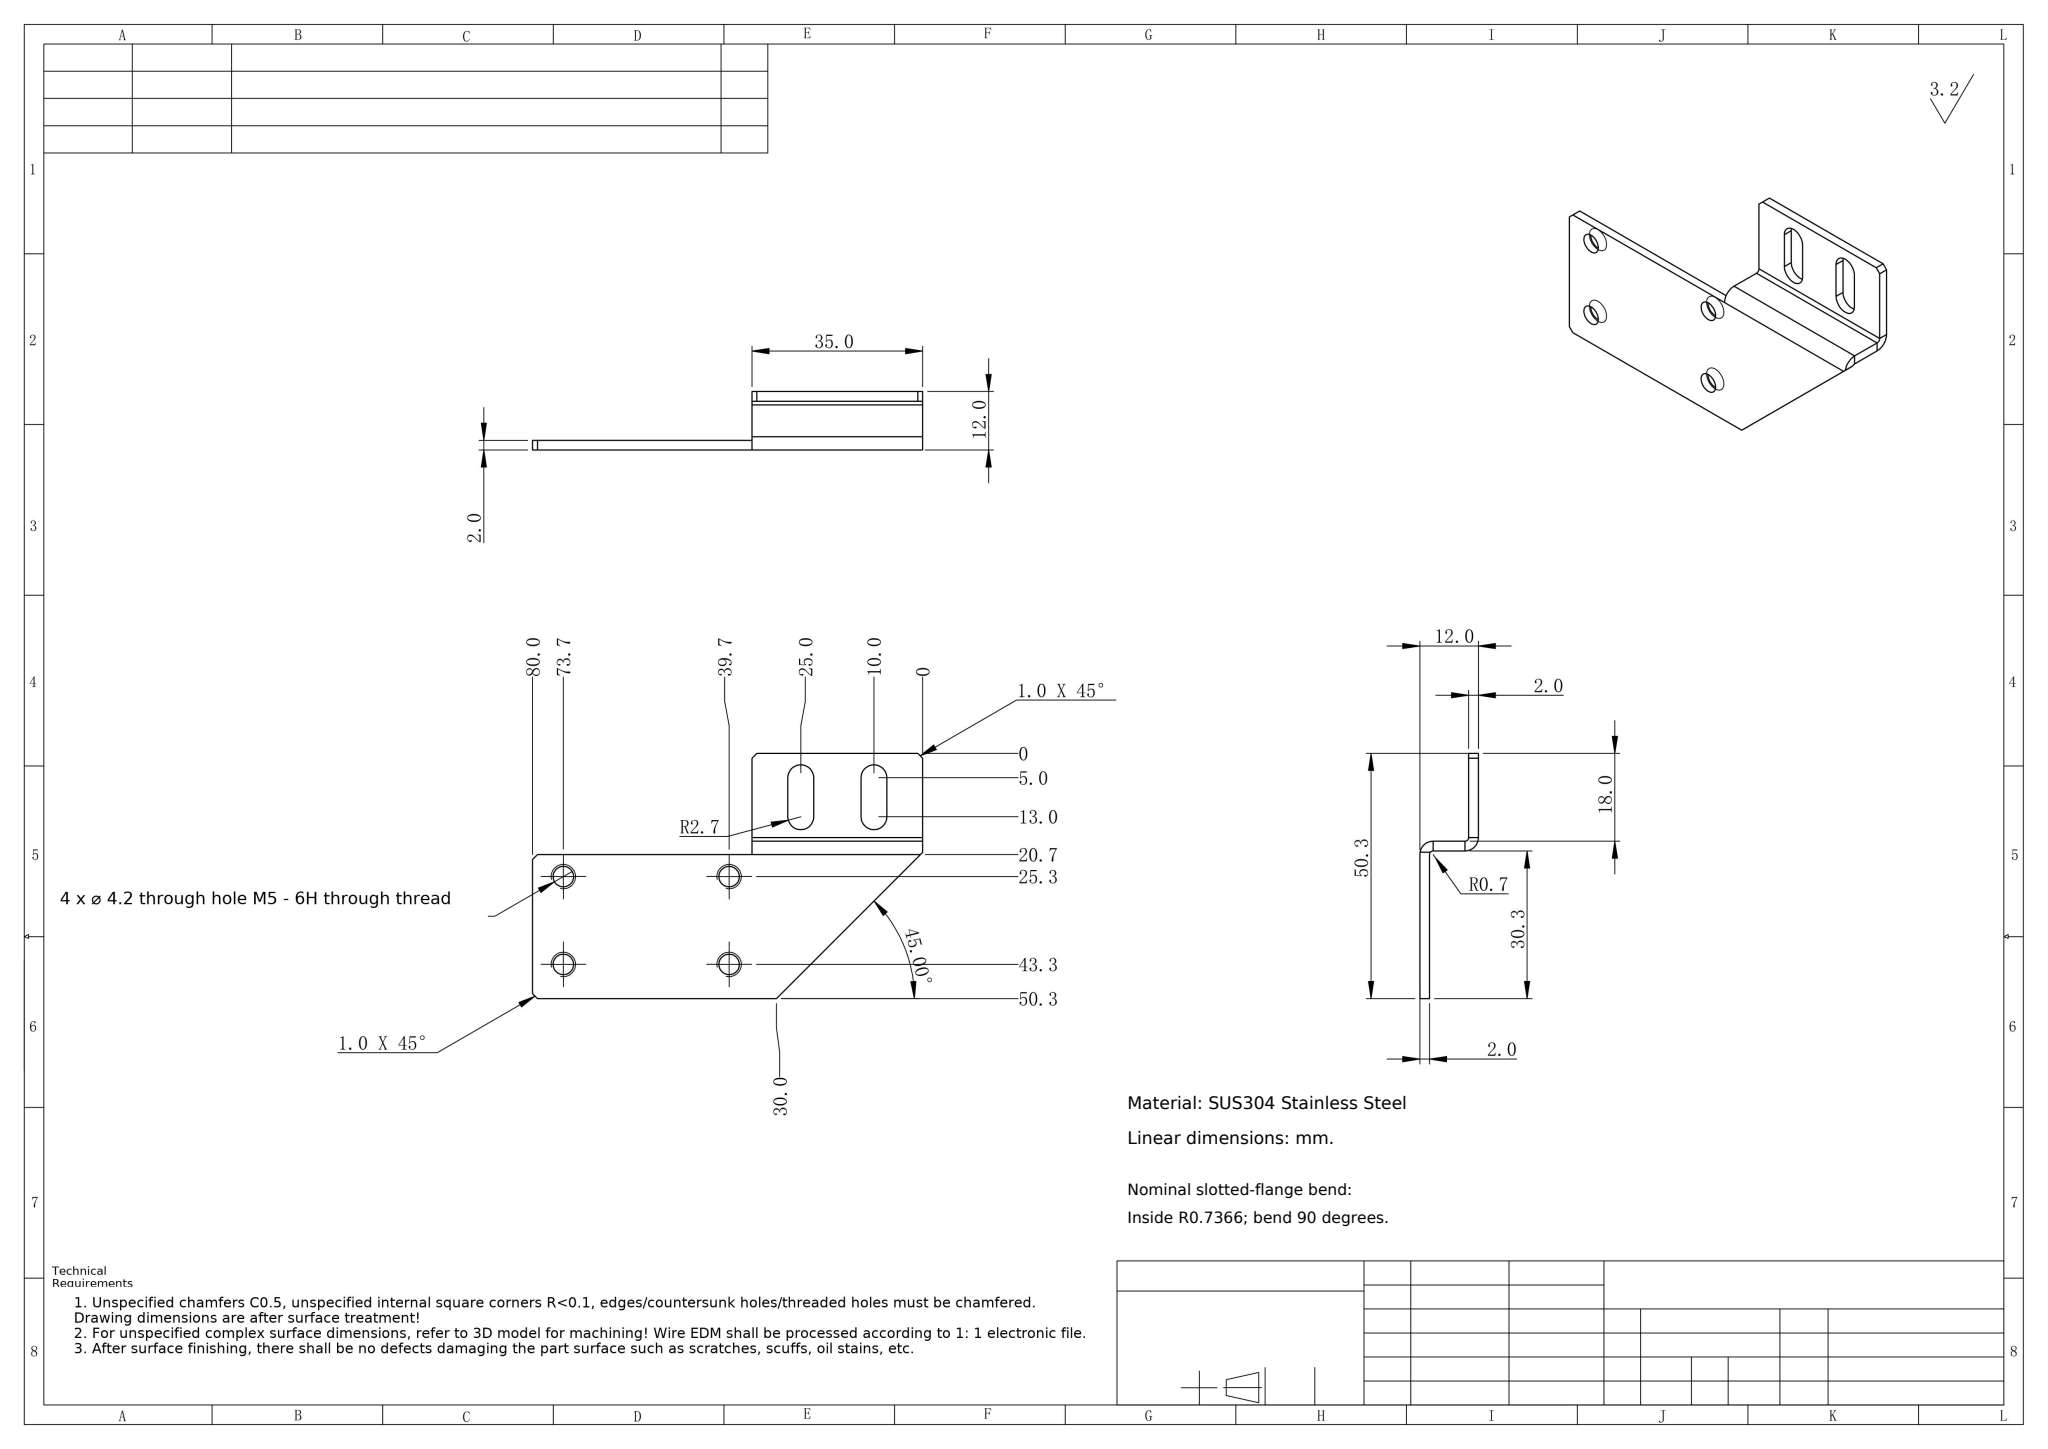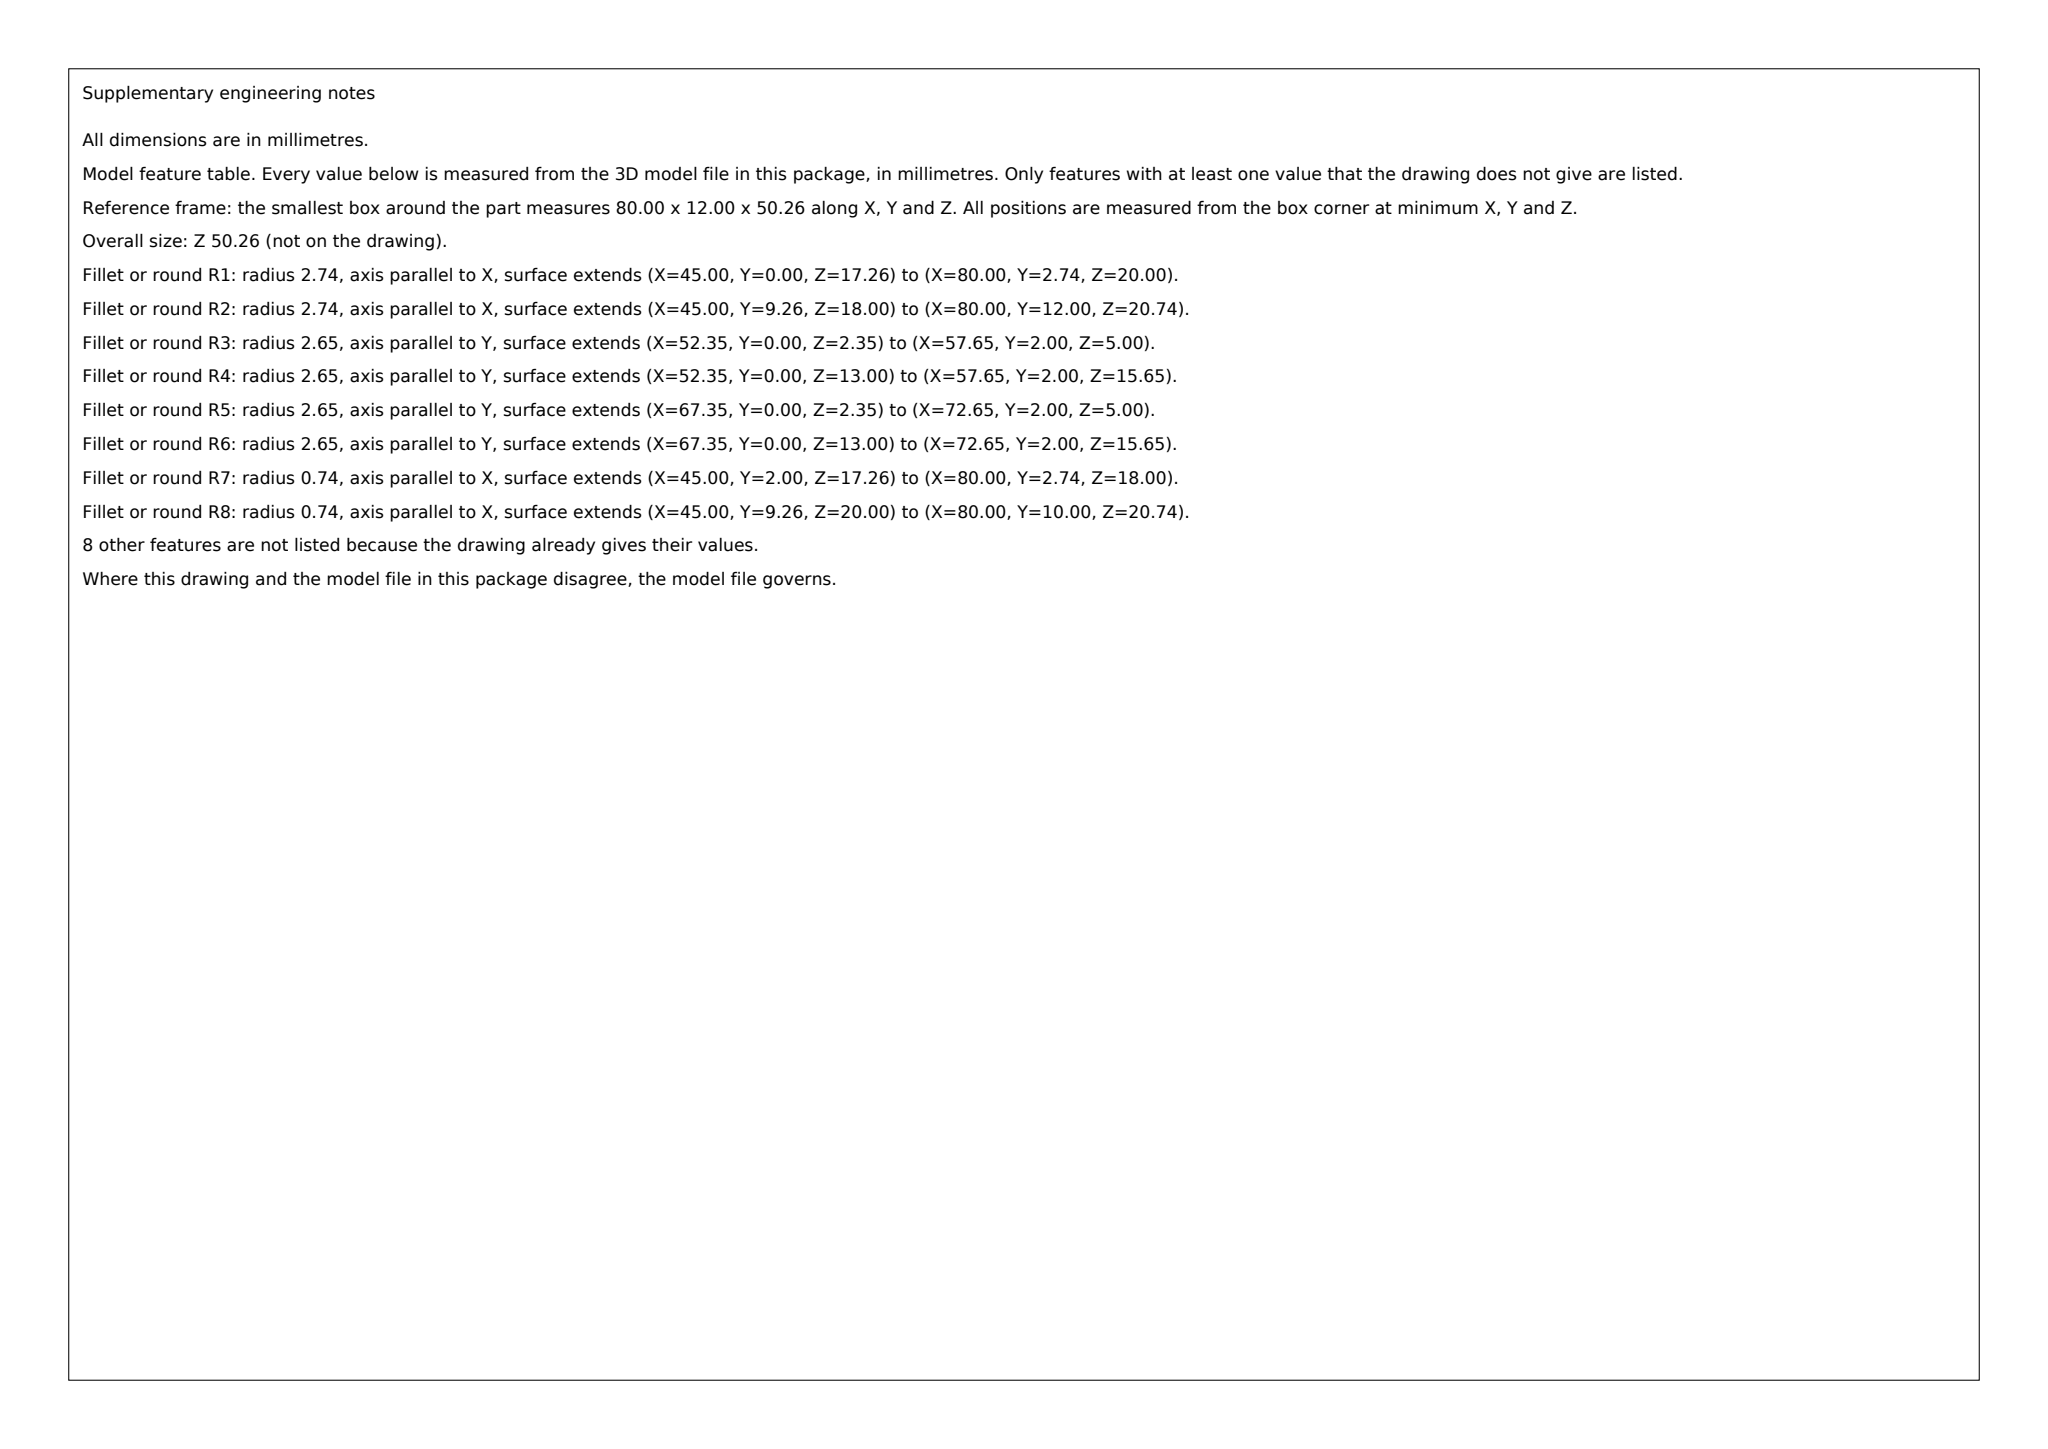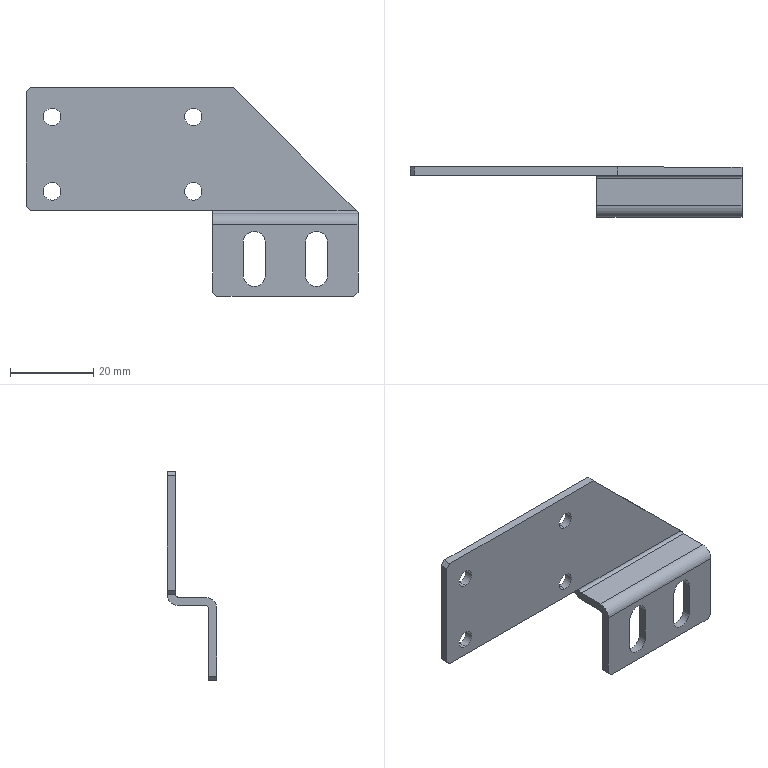Part | SolidWorks | mm | material SUS304 Stainless Steel | 1 solid | 42 faces | box 80 x 12 x 50.26 mm | volume 5499 mm3 | plane 24 | cylinder 18 | commonest cylinder face diameters 4.2 x8 5.3 x6 5.473 x2 1.473 x2